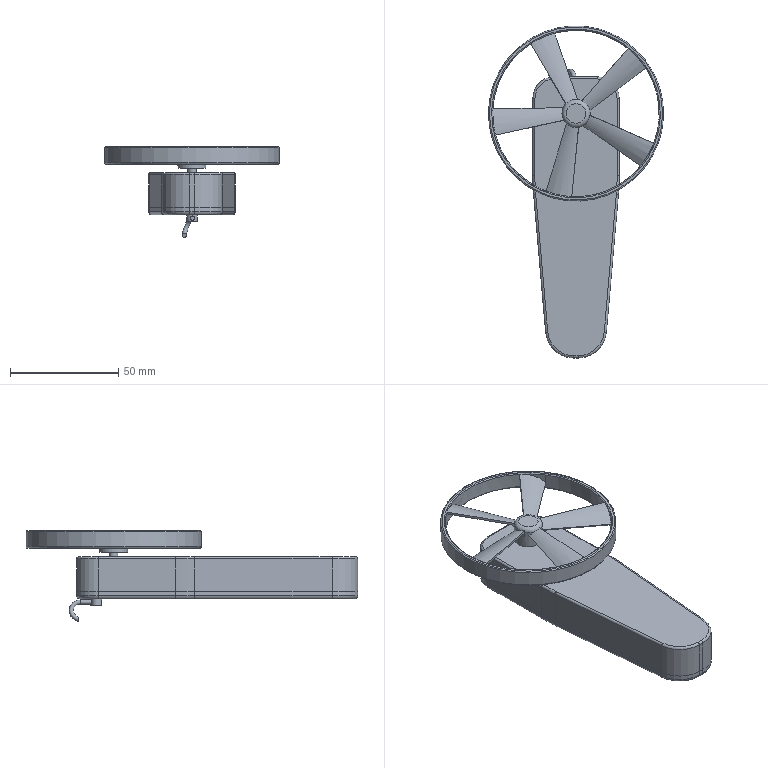Assembly | NX | mm | 10 component files | 10 solids | 1005 faces | box 81 x 153.5 x 41.84 mm | volume 54874 mm3 | other 465 | cylinder 244 | spline 165 | plane 103 | torus 19 | cone 9 | commonest cylinder face diameters 3 x36 25.5 x28 25.48 x28 23.5 x26 13.5 x16 12.5 x15 4 x9 196 x8
Bill of materials:
unnamed part 1 | 1 |  | Solid round rod bent into a J or hook shape: a long straight leg running into a tight bend of about 180 degrees that ends in a short return leg.
unnamed part 2 | 1 |  | Flat spur gear with straight teeth (roughly 28-30 of them) around the rim and a small round bore at the center.
unnamed part 3 | 1 |  | Tapered, paddle-shaped solid plate with rounded ends and edges, a small through hole near the wide end, and small pins sticking out of the underside.
unnamed part 4 | 1 |  | Spur gear with about 16 straight teeth and a fairly large central round bore. It is thicker than it is wide in proportion to its tooth size.
unnamed part 5 | 1 |  | Flanged cylindrical cap or plug: a thin circular flange with rounded edges sits on top of a cylindrical body, which has a round cross hole running through it.
unnamed part 6 | 1 |  | Compound gear cluster on a shaft: a larger spur gear and a smaller coaxial spur gear stacked together, with a shaft sticking out above the small gear and a short stub below the large gear.
unnamed part 7 | 1 |  | Short solid disc with a smaller coaxial cylindrical stem sticking out of one face, giving a T-shaped profile like a knob or headed pin.
unnamed part 8 | 1 |  | Spur gear with about 28 teeth and a central bore, with a narrower coaxial toothed section (a pinion) below it, forming a two-stage gear.
unnamed part 9 | 1 |  | Ducted rotor or fan-like part: five tapered blades run from a central round hub out to a thin surrounding ring, and a short hub boss sticks out on one side.
unnamed part 10 | 1 |  | Shallow tapered tray or base plate with a raised perimeter rim, six small upright pins near the rim, one through hole near the wide end, and several small circular recesses in the floor.
Mates:
1. fix | Casing 1 component
2. touch align | Gear_1 1 face | Casing 1 face
3. touch align | Gear_2 1 face | Casing 1 face
4. touch align | Gear_2 1 face | Casing 1 face
5. touch align | Gear_3 1 face | Casing 1 face
6. distance | Gear_3 1 face | Gear_2 1 face
7. touch align | Gear_4 1 face | Casing 1 face
8. touch align | Gear_4 1 face | Gear_3 1 face
9. touch align | Motor_Diagram 1 face | Casing 1 face
10. touch align | Motor_Diagram 1 face | Casing 1 face
11. touch align | Casing_2 1 face | Casing 1 face
12. touch align | Gear_1 1 face | Casing_2 1 face
13. touch align | Fan_Blade 1 face | Gear_1 1 face
14. touch align | Fan_Blade 1 face | Gear_1 1 face
15. concentric | Connecting_Pin 1 arc | Casing_2 1 edge
16. concentric | Casing_2 1 edge | Casing 1 edge
17. concentric | Casing_2 1 edge | Casing 1 edge
18. touch align | Hook 1 face | Connecting_Pin 1 face
19. touch align | Hook 1 face | Connecting_Pin 1 face